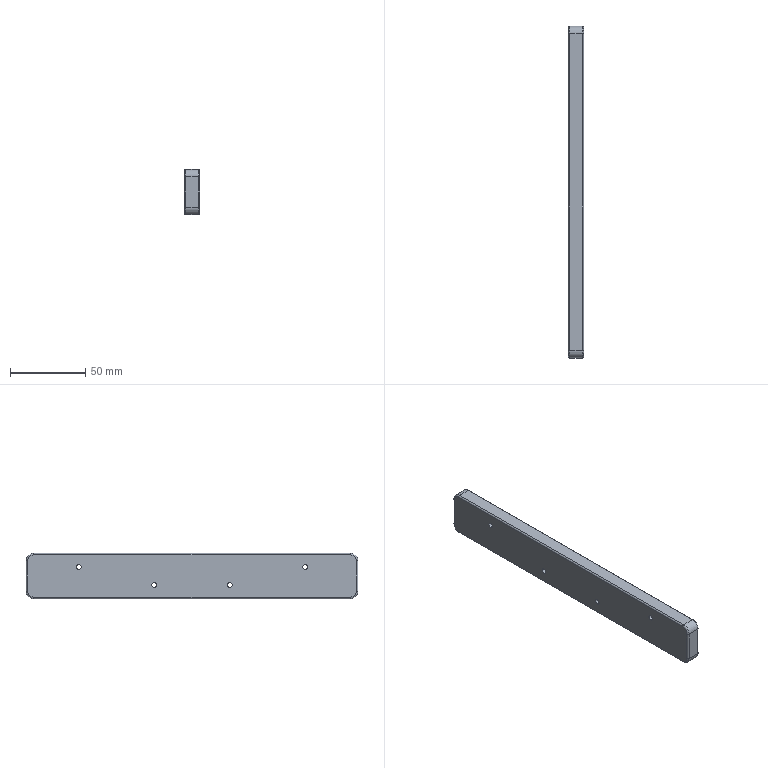CAM job | Mastercam | mm | 12 operations | part box 10 x 220 x 30
1. Facing | 23 - 50 平铣刀
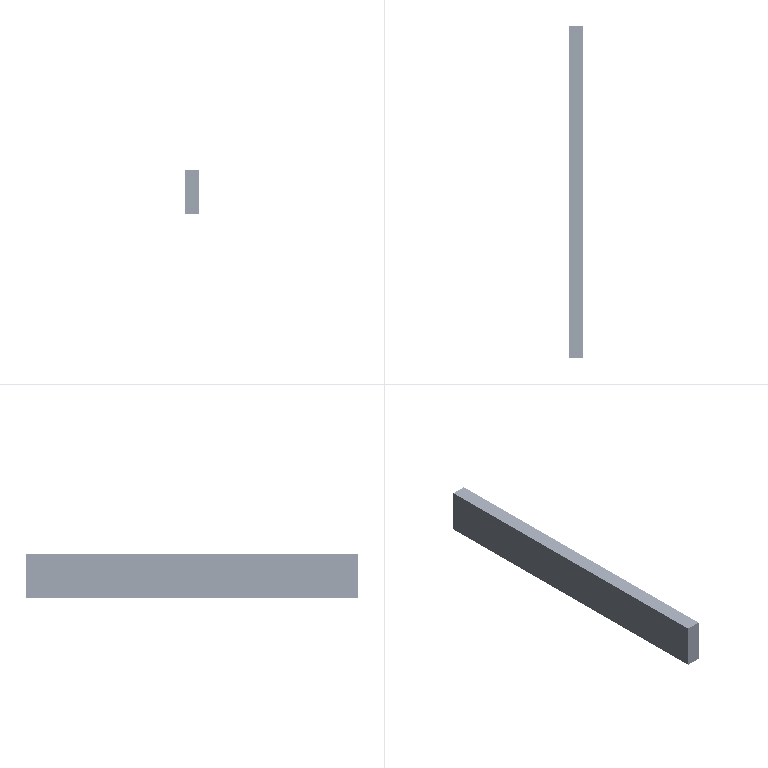2. Facing | 10 - 10 平铣刀
3. Contour (Ramp) | 9 - 10 平铣刀
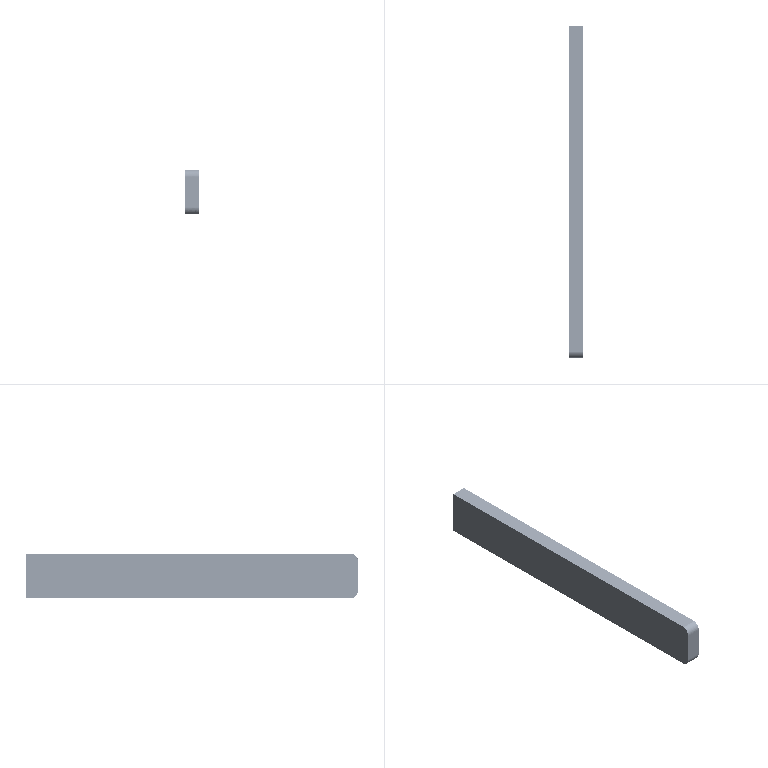4. Contour (Ramp) | 9 - 10 平铣刀
5. Contour (2D) | 10 - 10 平铣刀
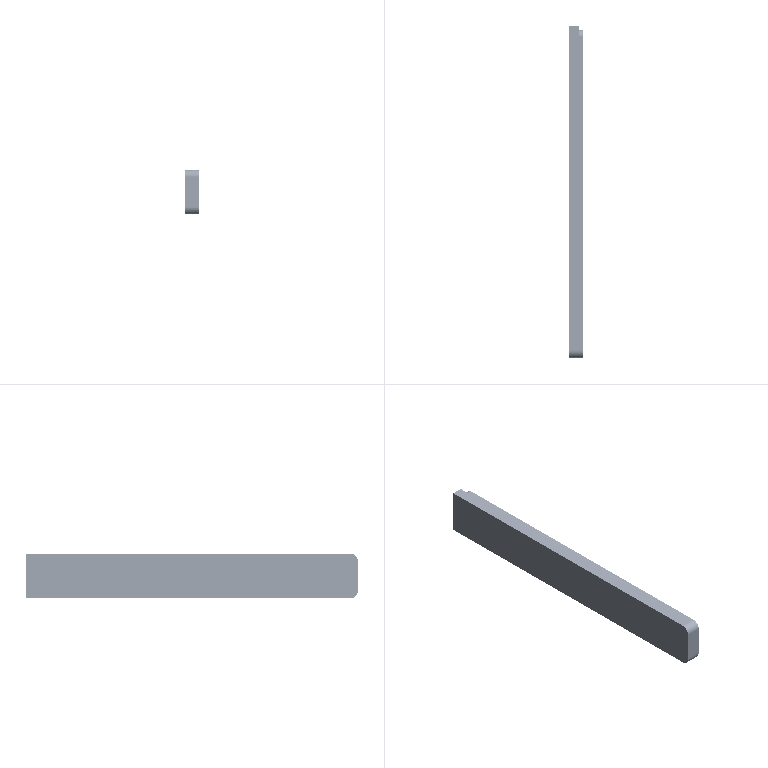6. Unified Morph | 18 - 10 圆鼻铣刀
7. Drill/Counterbore | 7 - 6 倒角刀
8. Facing | 23 - 50 平铣刀
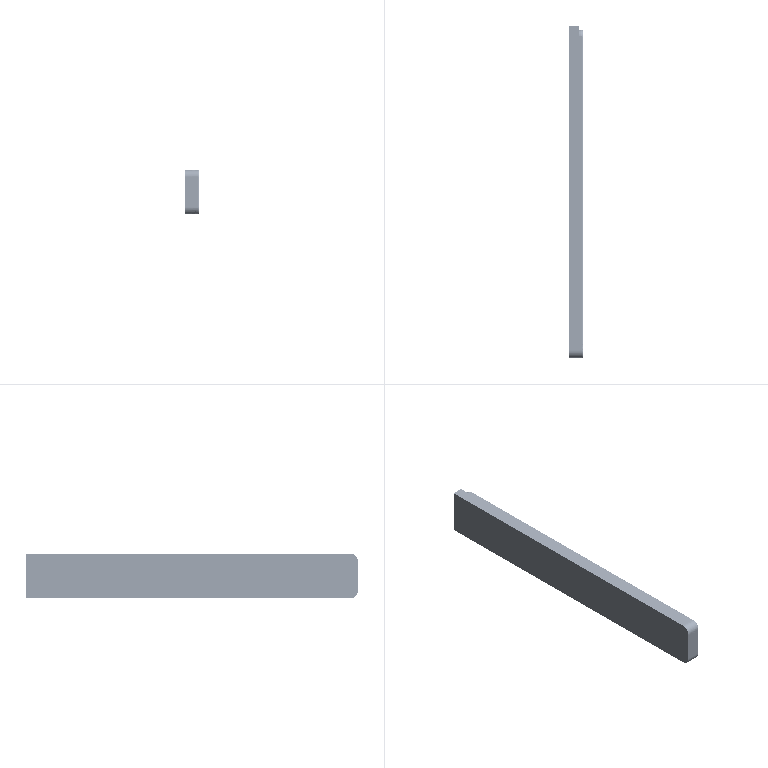9. Facing | 10 - 10 平铣刀
10. Contour (Ramp) | 9 - 10 平铣刀
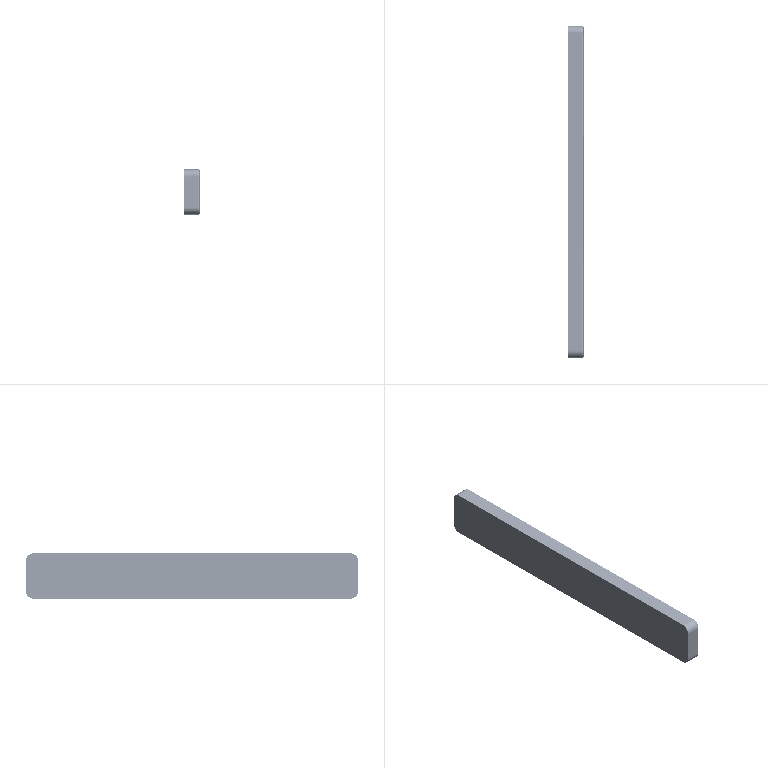11. Contour (2D) | 10 - 10 平铣刀
12. Unified Morph | 18 - 10 圆鼻铣刀